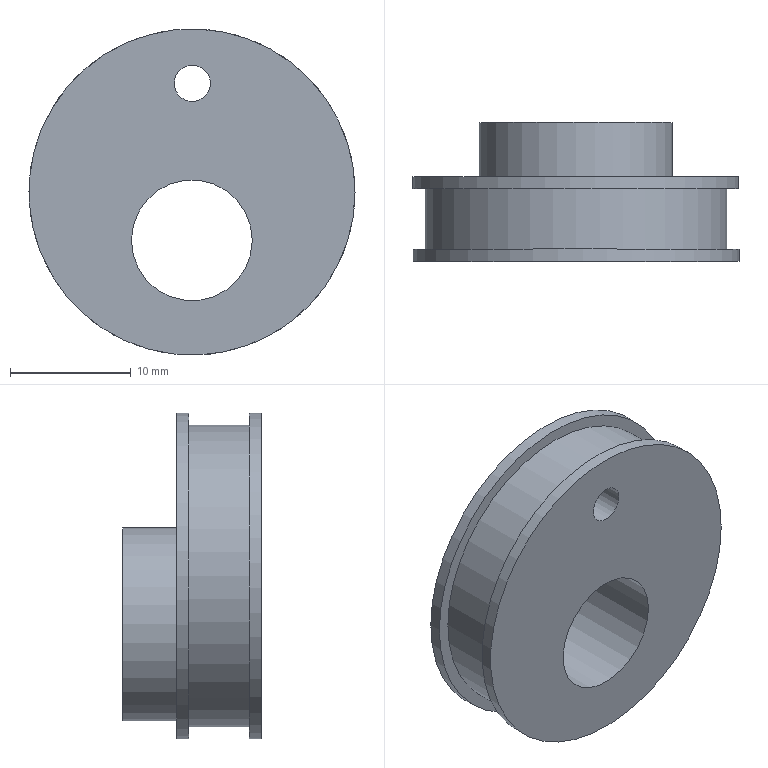Component | NX | ECCENTRIC_CAM | 1 solid | 11 faces | volume 3552 mm3 | cylinder 6 | plane 5 | commonest cylinder face diameters 27 x2 25 x1 16 x1 10 x1 3 x1